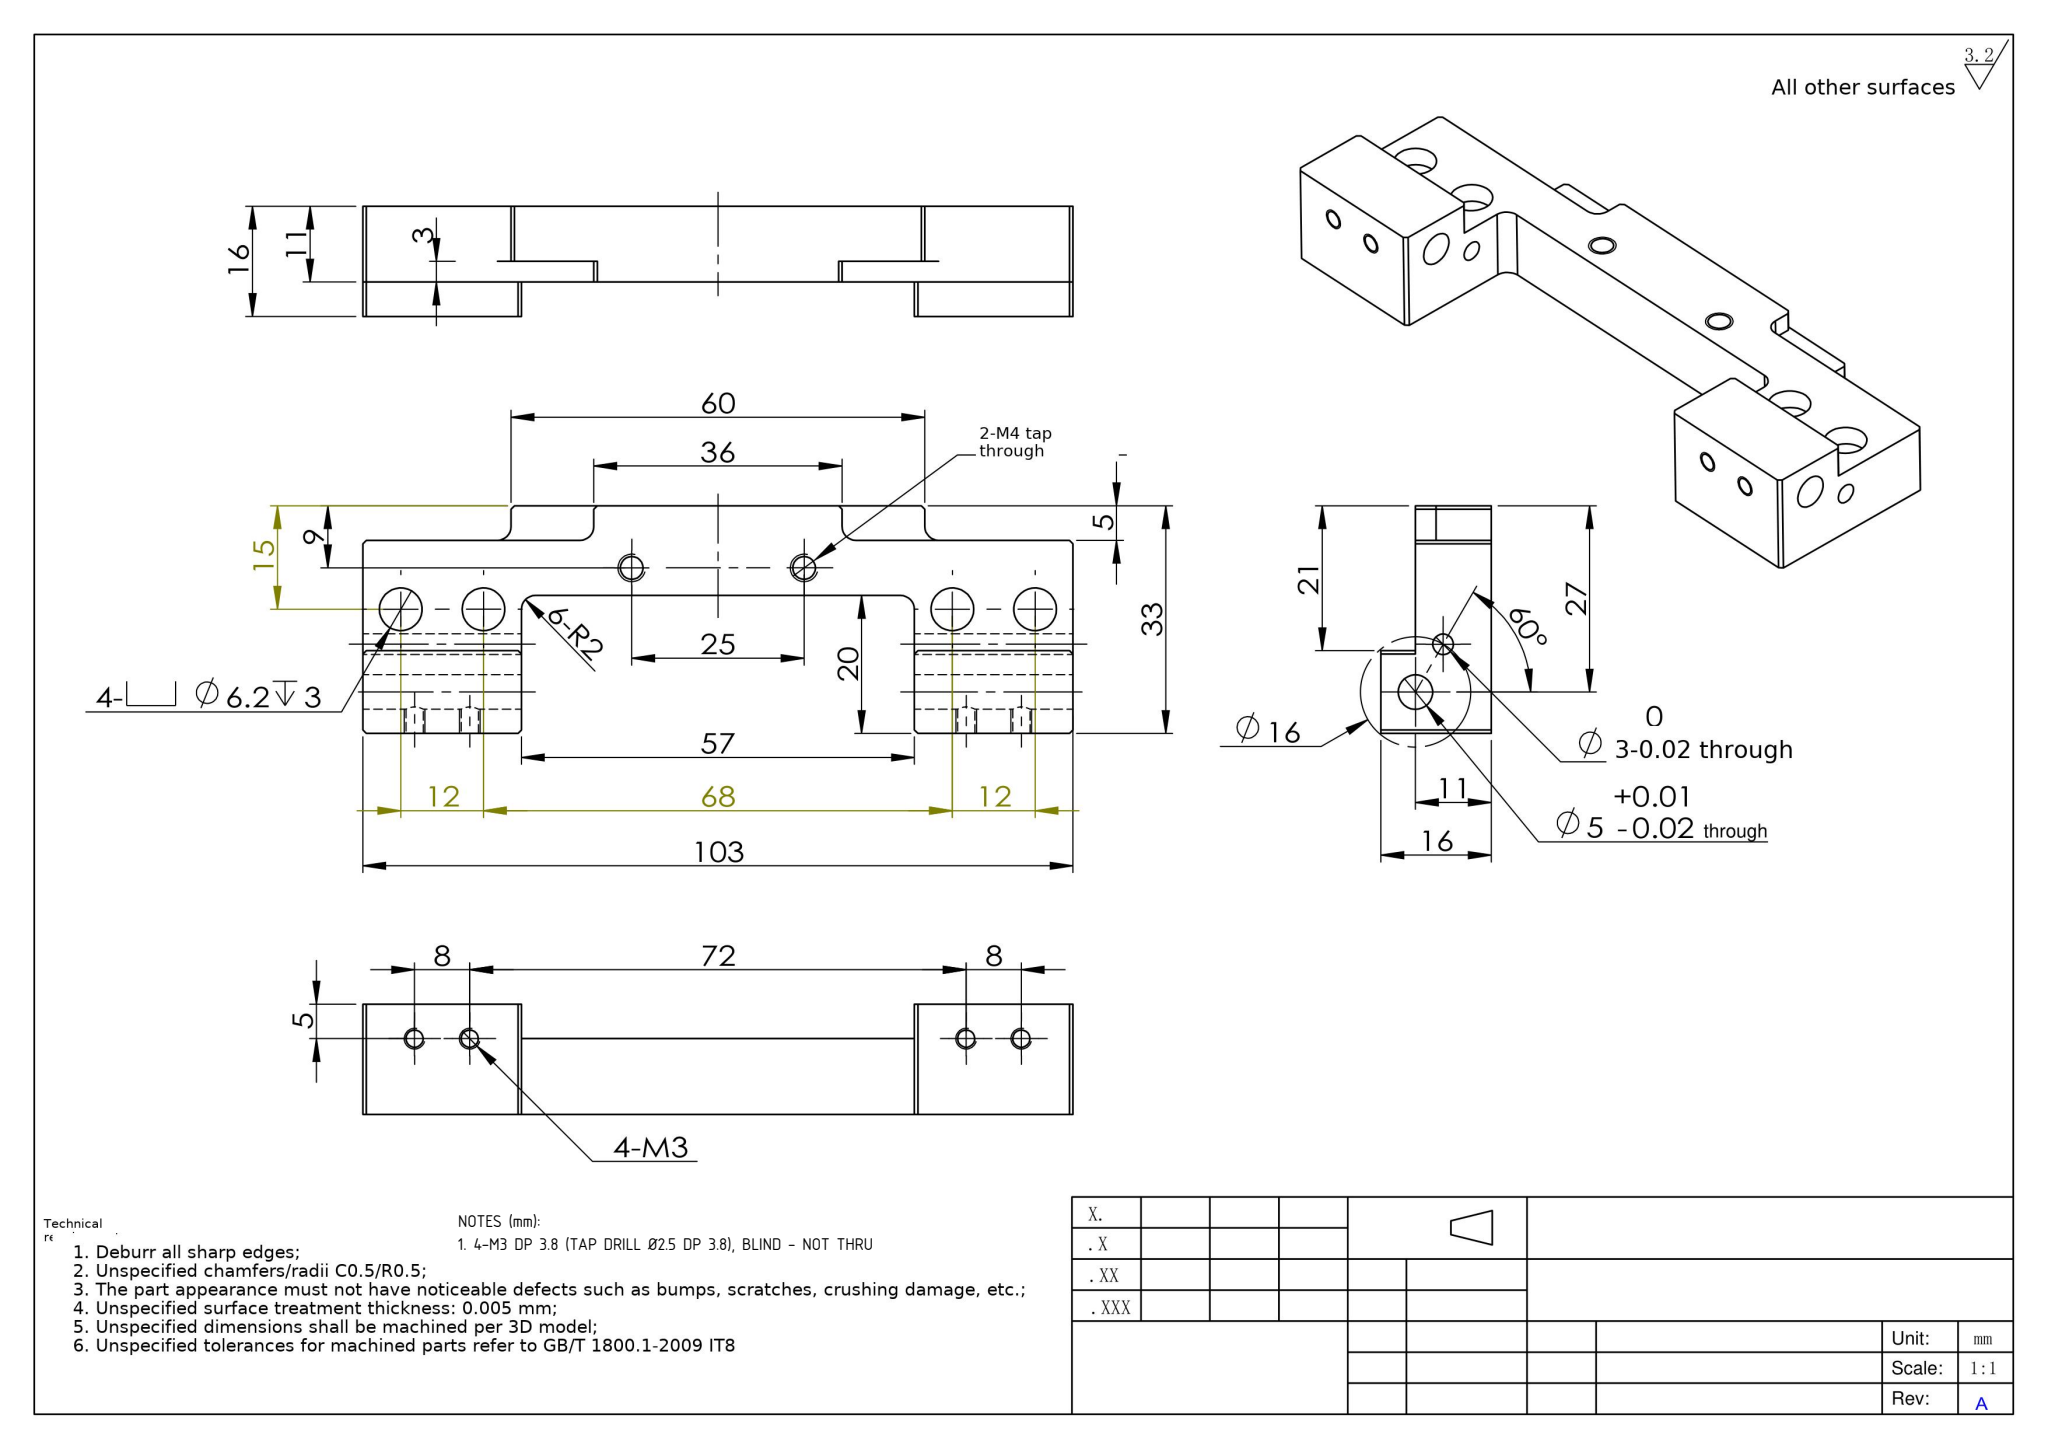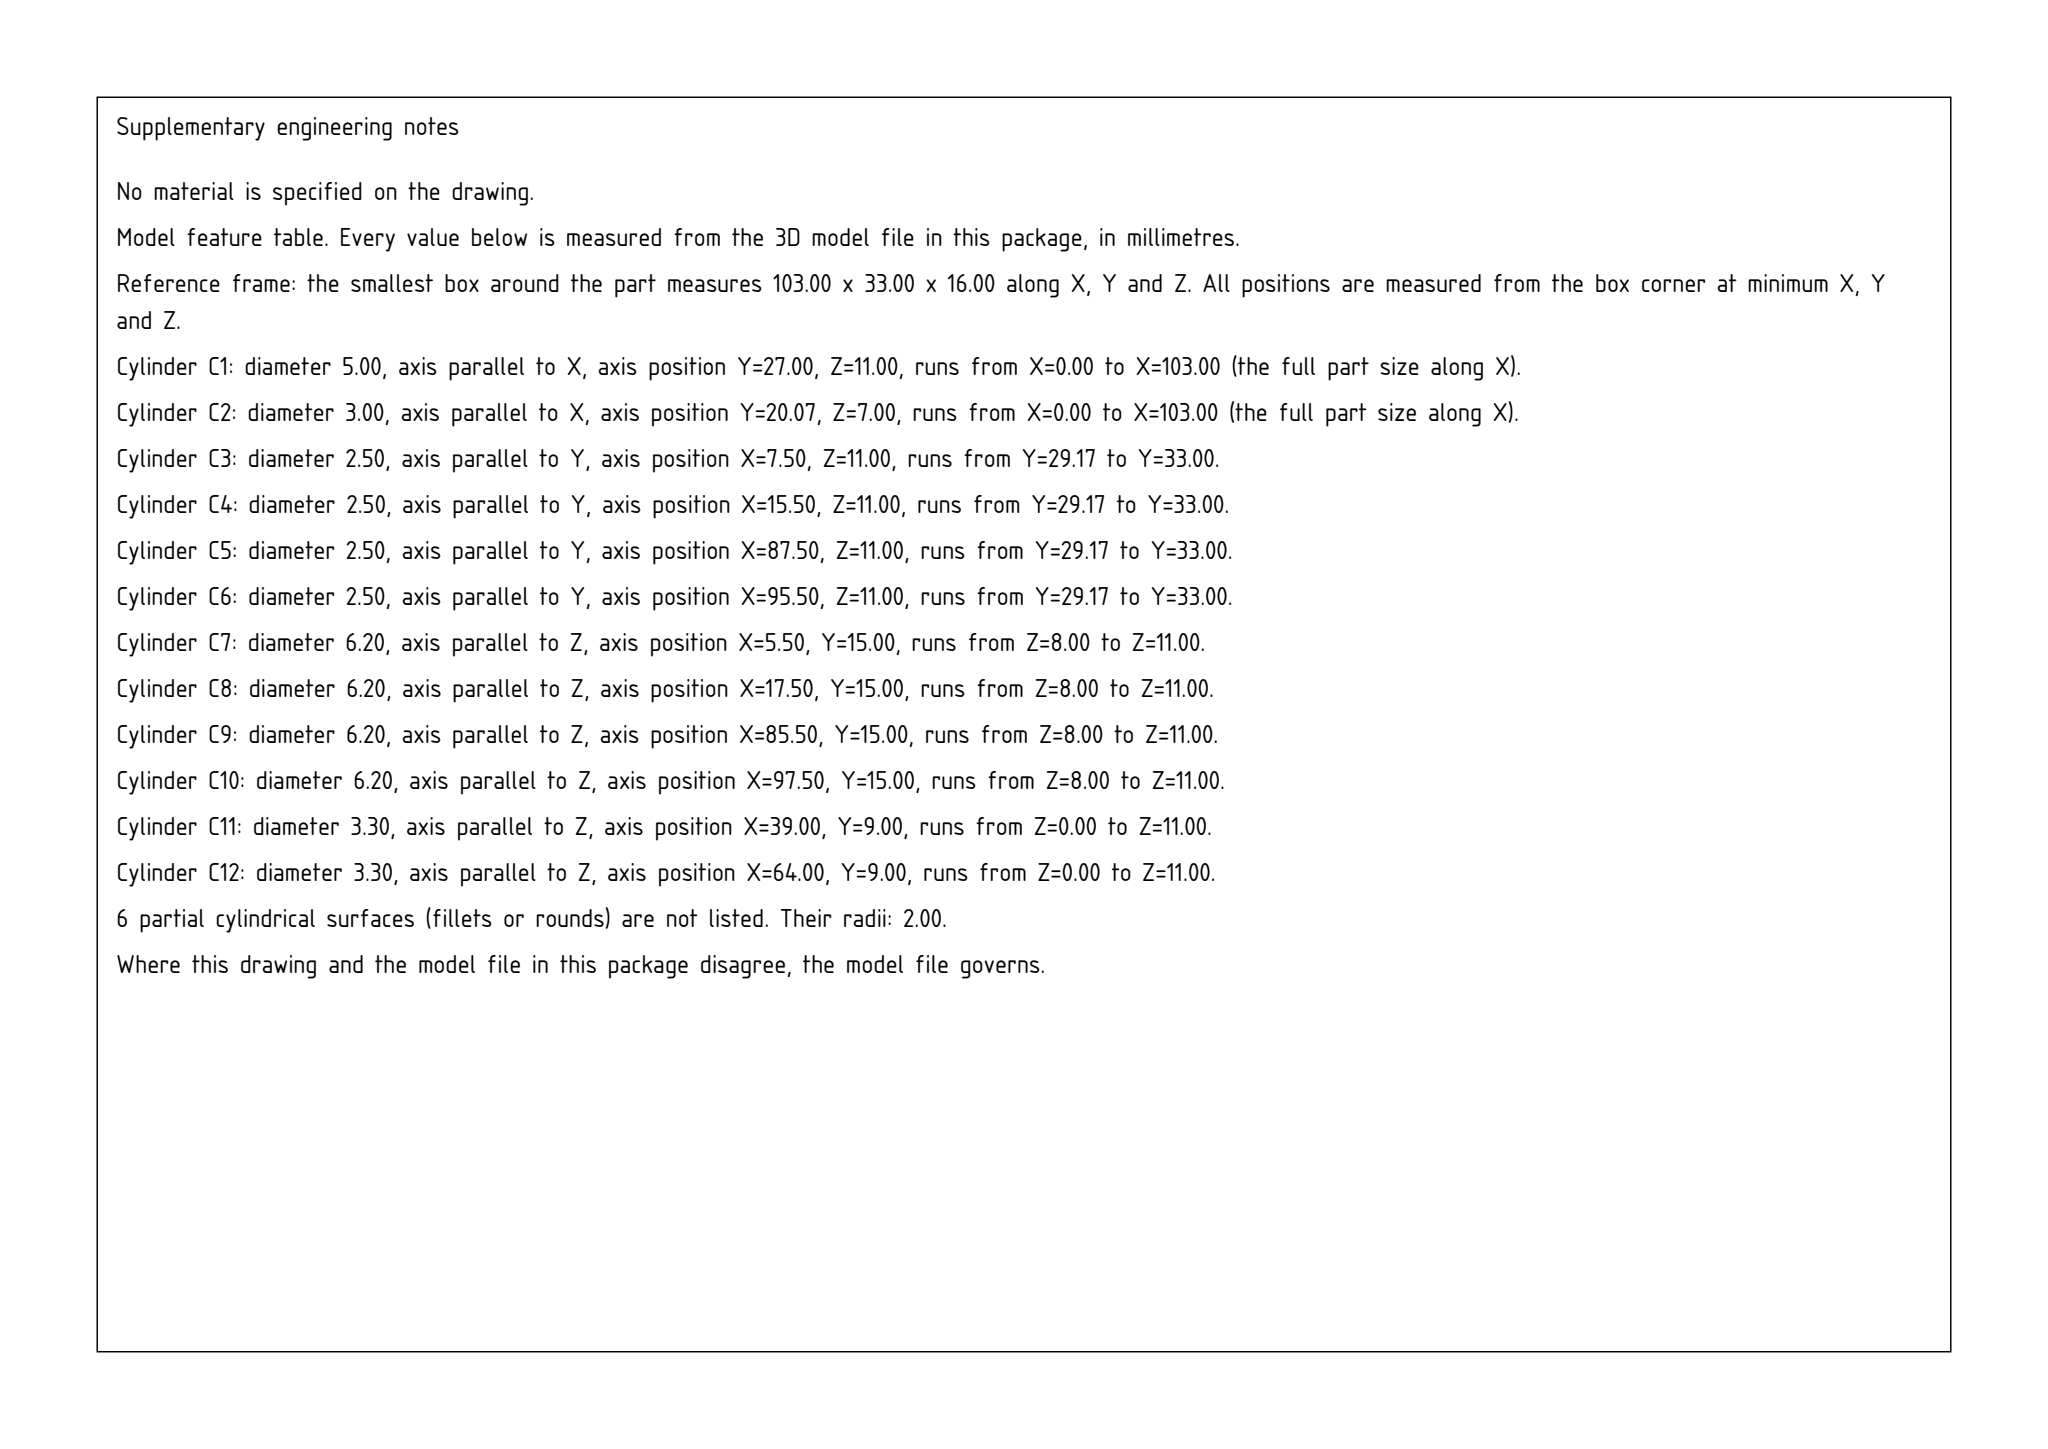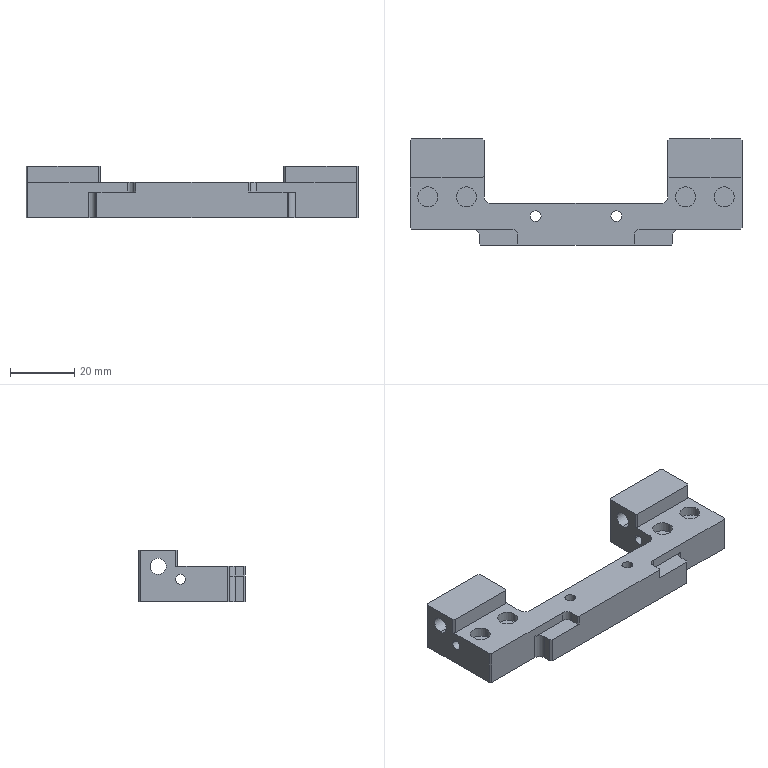Part | SolidWorks | mm | 1 solid | 74 faces | box 103 x 33 x 16 mm | volume 23057 mm3 | plane 40 | cylinder 34 | commonest cylinder face diameters 2.5 x8 6.2 x8 4 x6 3.3 x4 3 x4 5 x4
Drawing notes:
4-M3 DP 3.8 (TAP DRILL Ø2.5 DP 3.8), BLIND - NOT THRU | from the solid: 4x Ø2.5 cyl, axis y, at x=7.5/15.5/87.5/95.5, z=11.0, length 3.83 from y=0 face
build123d program:
from build123d import *

# Parameters (mm, degrees)
SKETCH1_W              = 103
SKETCH1_H              = 28
BOSS_EXTRUDE1_DEPTH    = 8
SKETCH2_W              = 9.5
SKETCH2_H              = 20
CUT_EXTRUDE1_DEPTH     = 56.716
SKETCH19_W             = 23
SKETCH19_H             = 16
CUT_EXTRUDE8_DEPTH     = 5
SKETCH8_R              = 3.1
CUT_EXTRUDE5_DEPTH     = 8
SKETCH4_R              = 2.5
CUT_EXTRUDE2_DEPTH     = 23
CUT_EXTRUDE12_START    = -23
SKETCH26_R             = 2.5
CUT_EXTRUDE12_DEPTH    = 23
SKETCH25_R             = 1.5
CUT_EXTRUDE11_DEPTH    = 23
CUT_EXTRUDE13_START    = -23
SKETCH27_R             = 1.5
CUT_EXTRUDE13_DEPTH    = 23
M3_TAPPED_HOLE1_REACH  = 61.163
M3_TAPPED_HOLE1_BORE_R = 1.25
SKETCH28_W             = 57
SKETCH28_H             = 28
CUT_EXTRUDE14_DEPTH    = 5
M4_TAPPED_HOLE1_D      = 3.3
SKETCH32_W             = 38
SKETCH32_H             = 20
CUT_EXTRUDE15_DEPTH    = 55.491
SKETCH33_W             = 60
SKETCH33_H             = 11
BOSS_EXTRUDE2_DEPTH    = 5
CUT_EXTRUDE16_DEPTH    = 3
FILLET1_R              = 2
CHAMFER1_SIZE          = 0.5


with BuildPart() as part:
    # Sketch1 → Boss-Extrude1 (new, symmetric)
    with BuildSketch(Plane.XY):
        Rectangle(SKETCH1_W, SKETCH1_H)
    extrude(amount=BOSS_EXTRUDE1_DEPTH, both=True)

    # Sketch2 → Cut-Extrude1 (cut, through all)
    with BuildSketch(Plane(origin=(0, 0, -8), x_dir=(-1, 0, 0), z_dir=(0, 0, -1))):
        with Locations((23.75, 4)):
            Rectangle(SKETCH2_W, SKETCH2_H)
        with Locations((-23.75, 4)):
            Rectangle(SKETCH2_W, SKETCH2_H)
    extrude(amount=-CUT_EXTRUDE1_DEPTH, mode=Mode.SUBTRACT)

    # Sketch19 → Cut-Extrude8 (cut)
    with BuildSketch(Plane.XY.offset(8)):
        with Locations((-40, -6)):
            Rectangle(SKETCH19_W, SKETCH19_H)
        with Locations((40, -6)):
            Rectangle(SKETCH19_W, SKETCH19_H)
    extrude(amount=-CUT_EXTRUDE8_DEPTH, mode=Mode.SUBTRACT)

    # Sketch8 → Cut-Extrude5 (cut)
    with BuildSketch(Plane.XY.offset(8)):
        with Locations((46, -4)):
            Circle(SKETCH8_R)
        with Locations((34, -4)):
            Circle(SKETCH8_R)
        with Locations((-34, -4)):
            Circle(SKETCH8_R)
        with Locations((-46, -4)):
            Circle(SKETCH8_R)
    extrude(amount=-CUT_EXTRUDE5_DEPTH, mode=Mode.SUBTRACT)

    # Sketch4 → Cut-Extrude2 (cut)
    with BuildSketch(Plane.ZY.offset(51.5)):
        with Locations((3, 8)):
            Circle(SKETCH4_R)
    extrude(amount=-CUT_EXTRUDE2_DEPTH, mode=Mode.SUBTRACT)

    # Sketch26 → Cut-Extrude12 (cut)
    with BuildSketch(Plane(origin=(51.5, 0, 0), x_dir=(0, 0, -1), z_dir=(1, 0, 0)).offset(CUT_EXTRUDE12_START)):
        with Locations(Location((-3, 8, 0), (0, 0, 180))):
            Circle(SKETCH26_R)
    extrude(amount=CUT_EXTRUDE12_DEPTH, mode=Mode.SUBTRACT)

    # Sketch25 → Cut-Extrude11 (cut)
    with BuildSketch(Plane(origin=(51.5, 0, 0), x_dir=(0, 0, -1), z_dir=(1, 0, 0))):
        with Locations(Location((1, 1.072, 0), (0, 0, 90))):
            Circle(SKETCH25_R)
    extrude(amount=-CUT_EXTRUDE11_DEPTH, mode=Mode.SUBTRACT)

    # Sketch27 → Cut-Extrude13 (cut)
    with BuildSketch(Plane.ZY.offset(51.5).offset(CUT_EXTRUDE13_START)):
        with Locations(Location((-1, 1.072, 0), (0, 0, 90))):
            Circle(SKETCH27_R)
    extrude(amount=CUT_EXTRUDE13_DEPTH, mode=Mode.SUBTRACT)

    # M3 Tapped Hole1 bore → M3 Tapped Hole1 (cut, up to next)
    with BuildSketch(Plane(origin=(0, 14, 0), x_dir=(1, 0, 0), z_dir=(0, 1, 0)), mode=Mode.PRIVATE) as m3_tapped_hole1_sk1:
        with Locations((36, -3)):
            Circle(M3_TAPPED_HOLE1_BORE_R)
    m3_tapped_hole1_tool1 = extrude(m3_tapped_hole1_sk1.sketch, amount=-M3_TAPPED_HOLE1_REACH, mode=Mode.PRIVATE) & part.part
    # M3 Tapped Hole1 bore → M3 Tapped Hole1 (cut, up to next)
    with BuildSketch(Plane(origin=(0, 14, 0), x_dir=(1, 0, 0), z_dir=(0, 1, 0)), mode=Mode.PRIVATE) as m3_tapped_hole1_sk2:
        with Locations((44, -3)):
            Circle(M3_TAPPED_HOLE1_BORE_R)
    m3_tapped_hole1_tool2 = extrude(m3_tapped_hole1_sk2.sketch, amount=-M3_TAPPED_HOLE1_REACH, mode=Mode.PRIVATE) & part.part
    # M3 Tapped Hole1 bore → M3 Tapped Hole1 (cut, up to next)
    with BuildSketch(Plane(origin=(0, 14, 0), x_dir=(1, 0, 0), z_dir=(0, 1, 0)), mode=Mode.PRIVATE) as m3_tapped_hole1_sk3:
        with Locations((-44, -3)):
            Circle(M3_TAPPED_HOLE1_BORE_R)
    m3_tapped_hole1_tool3 = extrude(m3_tapped_hole1_sk3.sketch, amount=-M3_TAPPED_HOLE1_REACH, mode=Mode.PRIVATE) & part.part
    # M3 Tapped Hole1 bore → M3 Tapped Hole1 (cut, up to next)
    with BuildSketch(Plane(origin=(0, 14, 0), x_dir=(1, 0, 0), z_dir=(0, 1, 0)), mode=Mode.PRIVATE) as m3_tapped_hole1_sk4:
        with Locations((-36, -3)):
            Circle(M3_TAPPED_HOLE1_BORE_R)
    m3_tapped_hole1_tool4 = extrude(m3_tapped_hole1_sk4.sketch, amount=-M3_TAPPED_HOLE1_REACH, mode=Mode.PRIVATE) & part.part
    add(m3_tapped_hole1_tool1.solids().sort_by_distance((36, 14, 3))[0], mode=Mode.SUBTRACT)
    add(m3_tapped_hole1_tool2.solids().sort_by_distance((44, 14, 3))[0], mode=Mode.SUBTRACT)
    add(m3_tapped_hole1_tool3.solids().sort_by_distance((-44, 14, 3))[0], mode=Mode.SUBTRACT)
    add(m3_tapped_hole1_tool4.solids().sort_by_distance((-36, 14, 3))[0], mode=Mode.SUBTRACT)

    # Sketch28 → Cut-Extrude14 (cut)
    with BuildSketch(Plane.XY.offset(8)):
        Rectangle(SKETCH28_W, SKETCH28_H)
    extrude(amount=-CUT_EXTRUDE14_DEPTH, mode=Mode.SUBTRACT)

    # M4 Tapped Hole1 (through all)
    with Locations(Plane.XY.offset(3)):
        with Locations((12.5, -10), (-12.5, -10)):
            Hole(M4_TAPPED_HOLE1_D / 2)

    # Sketch32 → Cut-Extrude15 (cut, through all)
    with BuildSketch(Plane.XY.offset(3)):
        with Locations((0, 4)):
            Rectangle(SKETCH32_W, SKETCH32_H)
    extrude(amount=-CUT_EXTRUDE15_DEPTH, mode=Mode.SUBTRACT)

    # Sketch33 → Boss-Extrude2 (add)
    with BuildSketch(Plane.XZ.offset(14)):
        with Locations((0, -2.5)):
            Rectangle(SKETCH33_W, SKETCH33_H)
    extrude(amount=BOSS_EXTRUDE2_DEPTH)

    # Sketch35 → Cut-Extrude16 (cut)
    with BuildSketch(Plane.XY.offset(3)):
        with BuildLine():
            Line((-30, -19), (-18, -19))
            Line((-18, -19), (-18, -16))
            ThreePointArc((-18, -16), (-18.586, -14.586), (-20, -14))
            Line((-20, -14), (-30, -14))
            Line((-30, -14), (-30, -19))
        make_face()
        with BuildLine():
            Line((30, -19), (18, -19))
            Line((18, -19), (18, -16))
            ThreePointArc((18, -16), (18.586, -14.586), (20, -14))
            Line((20, -14), (30, -14))
            Line((30, -14), (30, -19))
        make_face()
    extrude(amount=-CUT_EXTRUDE16_DEPTH, mode=Mode.SUBTRACT)

    # Fillet1
    fillet1_edges = [part.edges().sort_by_distance(p)[0] for p in [
        (28.5, -6, -2.5),
        (-28.5, -6, -2.5),
        (30, -14, -4),
        (-30, -14, -4),
    ]]
    fillet(fillet1_edges, radius=FILLET1_R)

    # Chamfer1
    chamfer1_edges = [part.edges().sort_by_distance(p)[0] for p in [
        (-51.5, 14, 0),
        (51.5, 14, 0),
        (-28.5, 14, 0),
        (51.5, 2, 5.5),
        (28.5, 14, 0),
        (28.5, 2, 5.5),
        (-28.5, 2, 5.5),
        (-51.5, 2, 5.5),
        (30, -19, -4),
        (-30, -19, -4),
        (18, -19, 1.5),
        (-18, -19, 1.5),
        (-51.5, -14, -2.5),
        (51.5, -14, -2.5),
    ]]
    chamfer(chamfer1_edges, length=CHAMFER1_SIZE)


solid = part.part